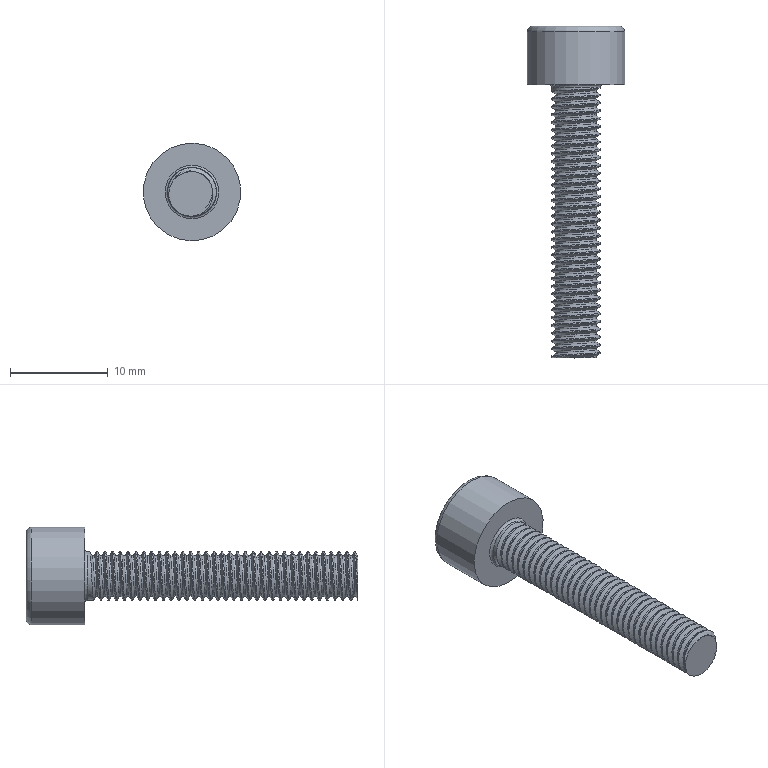Component | NX | M5X30_HEX_BOLT | 1 solid | 30 faces | volume 832 mm3 | plane 16 | cone 7 | cylinder 3 | torus 2 | spline 2 | commonest cylinder face diameters 5 x1 10 x1 4.2 x1